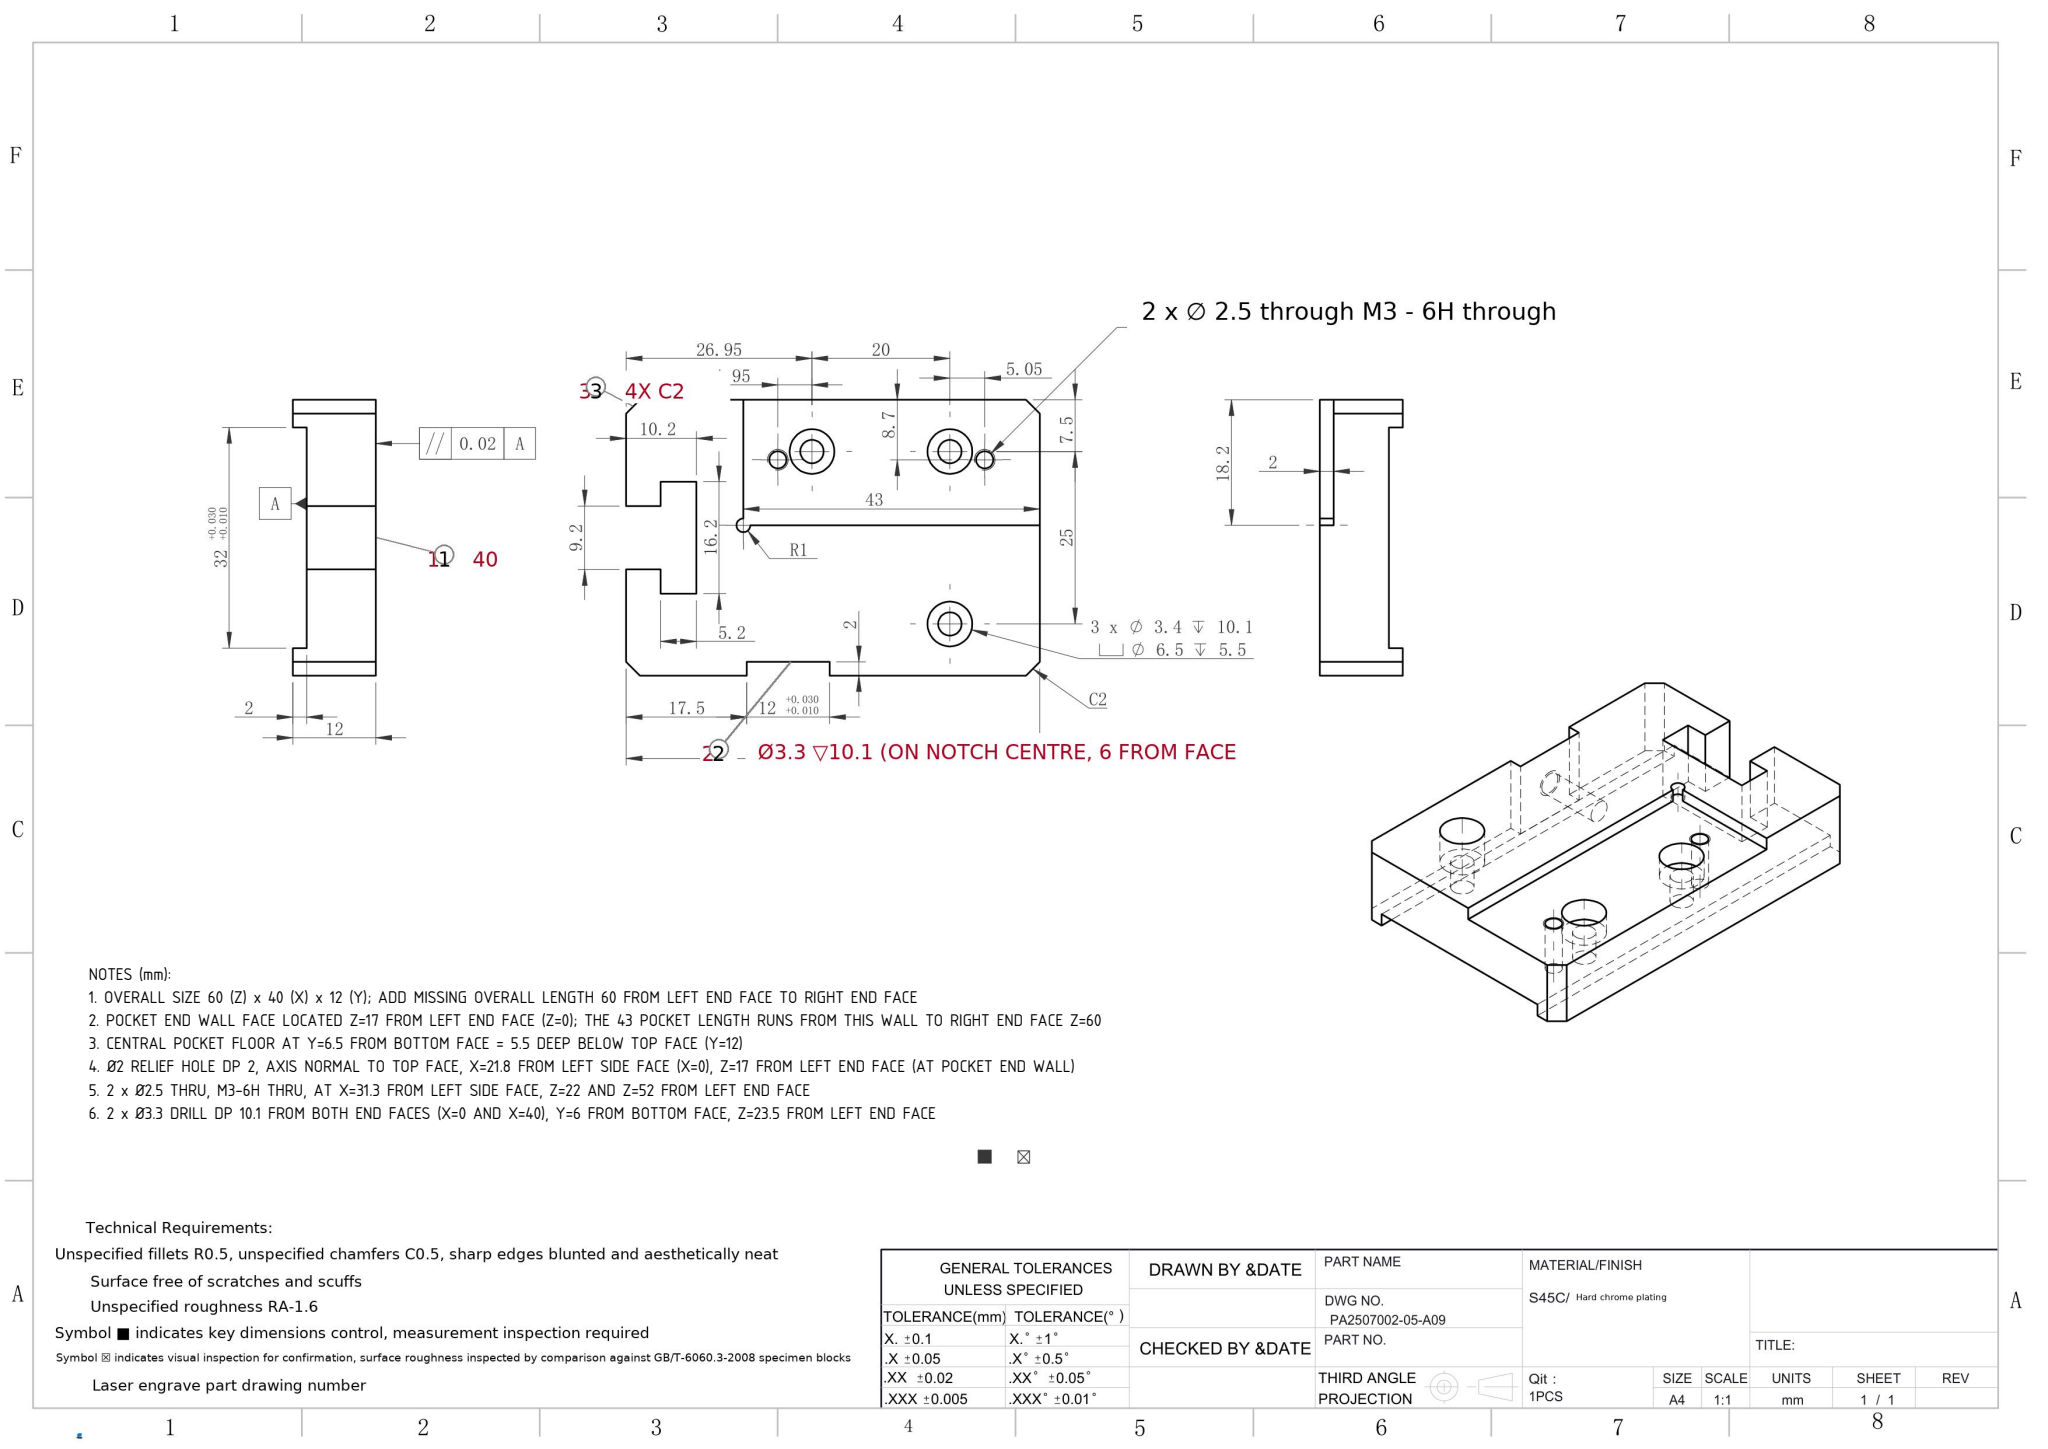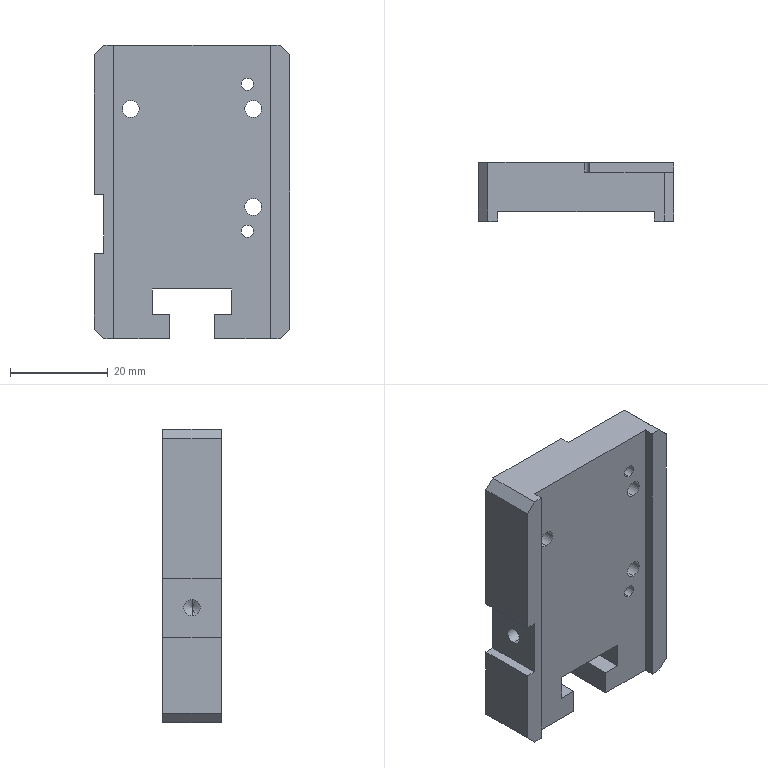Part | SolidWorks | mm | 1 solid | 53 faces | box 40 x 12 x 60 mm | volume 21003 mm3 | plane 32 | cylinder 19 | cone 2 | commonest cylinder face diameters 6.5 x6 3.4 x6 2.5 x4 3.3 x2 2 x1
Drawing notes:
OVERALL SIZE 60 (Z) x 40 (X) x 12 (Y); ADD MISSING OVERALL LENGTH 60 FROM LEFT END FACE TO RIGHT END FACE | from the solid: bbox_xyz [40.0, 12.0, 60.0]
POCKET END WALL FACE LOCATED Z=17 FROM LEFT END FACE (Z=0); THE 43 POCKET LENGTH RUNS FROM THIS WALL TO RIGHT END FACE Z=60 | from the solid: axis_planes z 17.0 and bbox z 60.0
CENTRAL POCKET FLOOR AT Y=6.5 FROM BOTTOM FACE = 5.5 DEEP BELOW TOP FACE (Y=12) | from the solid: axis_planes y 6.5 (3 faces) with bbox y 12.0
Ø2 RELIEF HOLE DP 2, AXIS NORMAL TO TOP FACE, X=21.8 FROM LEFT SIDE FACE (X=0), Z=17 FROM LEFT END FACE (AT POCKET END WALL) | from the solid: cylinder [2.0,"y",[21.8,null,17.0],2.0]
2 x Ø2.5 THRU, M3-6H THRU, AT X=31.3 FROM LEFT SIDE FACE, Z=22 AND Z=52 FROM LEFT END FACE | from the solid: cylinders [2.5,"y",[31.3,null,22.0]] and [2.5,"y",[31.3,null,52.0]]
2 x Ø3.3 DRILL DP 10.1 FROM BOTH END FACES (X=0 AND X=40), Y=6 FROM BOTTOM FACE, Z=23.5 FROM LEFT END FACE | from the solid: cylinder [3.3,"x",[null,6.0,23.5],10.1,2] with cone 118° ref dia 3.3
build123d program:
from build123d import *

# Parameters (mm, degrees)
SKETCH1_W                                       = 40
SKETCH1_H                                       = 12
BOSS_EXTRUDE1_DEPTH                             = 60
SKETCH2_W                                       = 32
SKETCH2_H                                       = 60
CUT_EXTRUDE1_DEPTH                              = 2
CUT_EXTRUDE2_DEPTH                              = 65.374
SKETCH4_W                                       = 12
SKETCH4_H                                       = 12
CUT_EXTRUDE3_DEPTH                              = 2
CHAMFER1_SIZE                                   = 2
M3_HEX_SOCKET_HEAD_CAP_SCREW_CBORE1_D           = 3.4
M3_HEX_SOCKET_HEAD_CAP_SCREW_CBORE1_DEPTH       = 10.1
M3_HEX_SOCKET_HEAD_CAP_SCREW_CBORE1_CBORE_D     = 6.5
M3_HEX_SOCKET_HEAD_CAP_SCREW_CBORE1_CBORE_DEPTH = 5.5
M3_HEX_SOCKET_HEAD_CAP_SCREW_CBORE1_TIP         = 1.021
M4_TAPPED_HOLE1_D                               = 3.3
M4_TAPPED_HOLE1_DEPTH                           = 10.1
M4_TAPPED_HOLE1_TIP                             = 0.9914
SKETCH10_W                                      = 18.2
SKETCH10_H                                      = 43
CUT_EXTRUDE4_DEPTH                              = 2
M3_TAPPED_HOLE1_D                               = 2.5
SKETCH13_R                                      = 1
CUT_EXTRUDE5_DEPTH                              = 2


with BuildPart() as part:
    # Sketch1 → Boss-Extrude1 (new body)
    with BuildSketch(Plane.XY):
        Rectangle(SKETCH1_W, SKETCH1_H)
    extrude(amount=BOSS_EXTRUDE1_DEPTH)

    # Sketch2 → Cut-Extrude1 (cut)
    with BuildSketch(Plane.XZ.offset(6)):
        with Locations((0, 30)):
            Rectangle(SKETCH2_W, SKETCH2_H)
    extrude(amount=-CUT_EXTRUDE1_DEPTH, mode=Mode.SUBTRACT)

    # Sketch3 → Cut-Extrude2 (cut, through all)
    with BuildSketch(Plane(origin=(0, 6, 0), x_dir=(1, 0, 0), z_dir=(0, 1, 0))):
        Polygon((4.6, 0), (4.6, -5), (8.1, -5), (8.1, -10.2), (-8.1, -10.2), (-8.1, -5), (-4.6, -5), (-4.6, 0), align=None)
    extrude(amount=-CUT_EXTRUDE2_DEPTH, mode=Mode.SUBTRACT)

    # Sketch4 → Cut-Extrude3 (cut)
    with BuildSketch(Plane.ZY.offset(20)):
        with Locations((23.5, 0)):
            Rectangle(SKETCH4_W, SKETCH4_H)
    extrude(amount=-CUT_EXTRUDE3_DEPTH, mode=Mode.SUBTRACT)

    # Chamfer1
    chamfer1_edges = [part.edges().sort_by_distance(p)[0] for p in [
        (-20, 0, 60),
        (20, 0, 60),
        (-20, 0, 0),
        (20, 0, 0),
    ]]
    chamfer(chamfer1_edges, length=CHAMFER1_SIZE)

    # M3 Hex Socket Head Cap Screw CBORE1
    with Locations(Plane(origin=(0, 6, 0), x_dir=(1, 0, 0), z_dir=(0, 1, 0))):
        with Locations((12.5, -26.95), (12.5, -46.95), (-12.5, -46.95)):
            CounterBoreHole(M3_HEX_SOCKET_HEAD_CAP_SCREW_CBORE1_D / 2, M3_HEX_SOCKET_HEAD_CAP_SCREW_CBORE1_CBORE_D / 2, M3_HEX_SOCKET_HEAD_CAP_SCREW_CBORE1_CBORE_DEPTH, depth=M3_HEX_SOCKET_HEAD_CAP_SCREW_CBORE1_DEPTH)
            with Locations((0, 0, -(M3_HEX_SOCKET_HEAD_CAP_SCREW_CBORE1_DEPTH + M3_HEX_SOCKET_HEAD_CAP_SCREW_CBORE1_TIP / 2))):  # 118° drill point
                Cone(0, M3_HEX_SOCKET_HEAD_CAP_SCREW_CBORE1_D / 2, M3_HEX_SOCKET_HEAD_CAP_SCREW_CBORE1_TIP, mode=Mode.SUBTRACT)

    # M4 Tapped Hole1
    with Locations(Plane.ZY.offset(18)):
        with Locations((23.5, 0)):
            Hole(M4_TAPPED_HOLE1_D / 2, depth=M4_TAPPED_HOLE1_DEPTH)
            with Locations((0, 0, -(M4_TAPPED_HOLE1_DEPTH + M4_TAPPED_HOLE1_TIP / 2))):  # 118° drill point
                Cone(0, M4_TAPPED_HOLE1_D / 2, M4_TAPPED_HOLE1_TIP, mode=Mode.SUBTRACT)

    # Sketch10 → Cut-Extrude4 (cut)
    with BuildSketch(Plane(origin=(0, 6, 0), x_dir=(1, 0, 0), z_dir=(0, 1, 0))):
        with Locations((10.9, -38.5)):
            Rectangle(SKETCH10_W, SKETCH10_H)
    extrude(amount=-CUT_EXTRUDE4_DEPTH, mode=Mode.SUBTRACT)

    # M3 Tapped Hole1 (through all)
    with Locations(Plane(origin=(0, 6, 0), x_dir=(1, 0, 0), z_dir=(0, 1, 0))):
        with Locations((11.3, -22), (11.3, -52)):
            Hole(M3_TAPPED_HOLE1_D / 2)

    # Sketch13 → Cut-Extrude5 (cut)
    with BuildSketch(Plane(origin=(0, 6, 0), x_dir=(1, 0, 0), z_dir=(0, 1, 0))):
        with Locations((1.8, -17)):
            Circle(SKETCH13_R)
    extrude(amount=-CUT_EXTRUDE5_DEPTH, mode=Mode.SUBTRACT)


solid = part.part